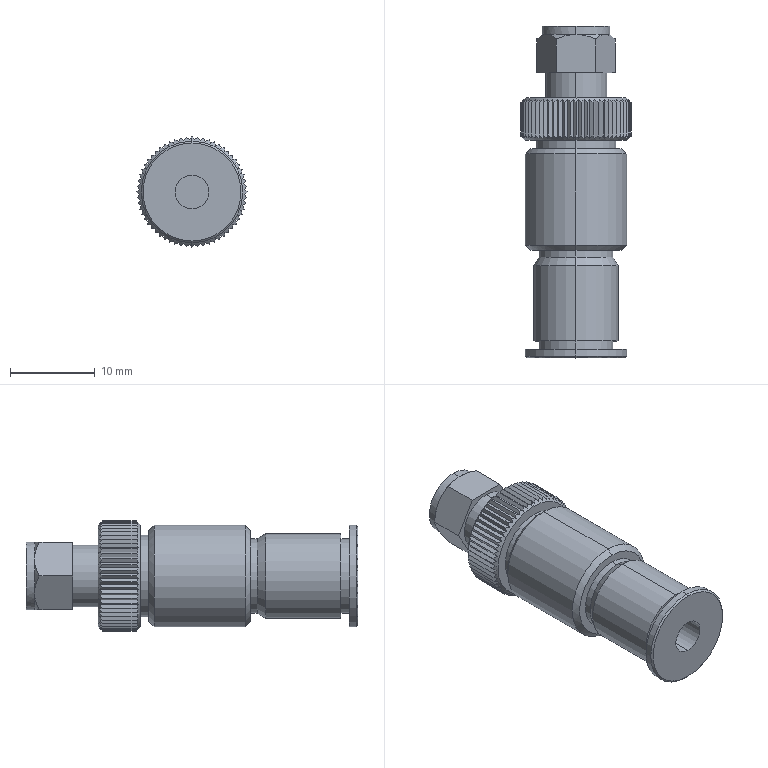Component | SolidWorks | HandlingMechanism-2_MVPTN2-1_1_2-1 | 1 solid | 175 faces | volume 3268 mm3 | plane 137 | cylinder 20 | cone 18 | commonest cylinder face diameters 12 x4 8.8 x4 4 x4 9.6 x2 10 x2 7.273 x2 8 x2